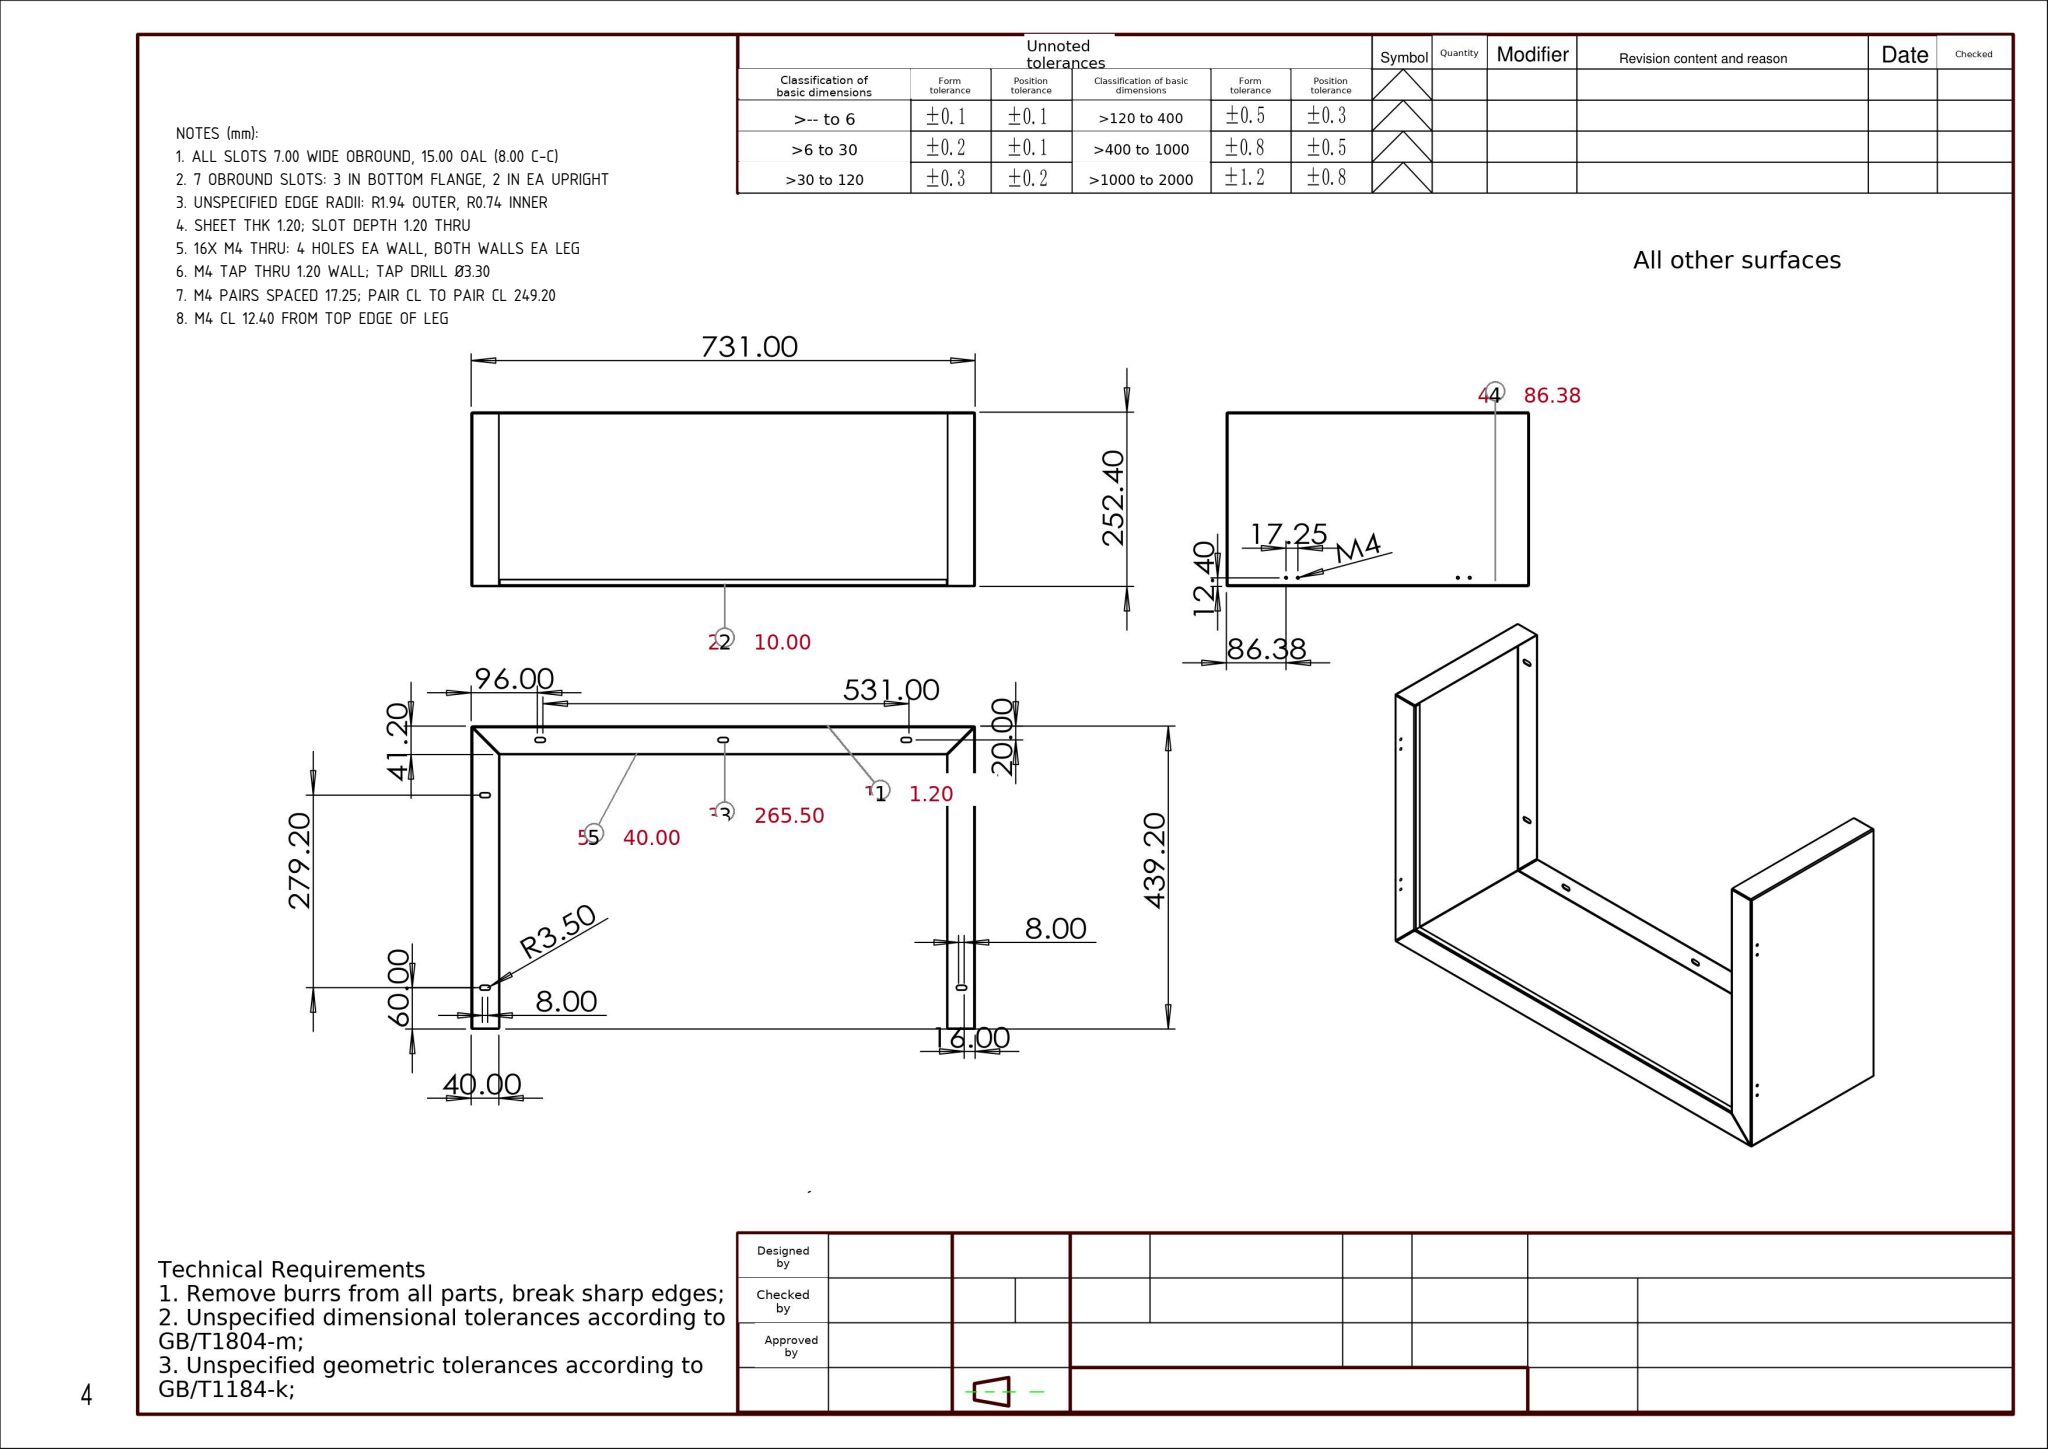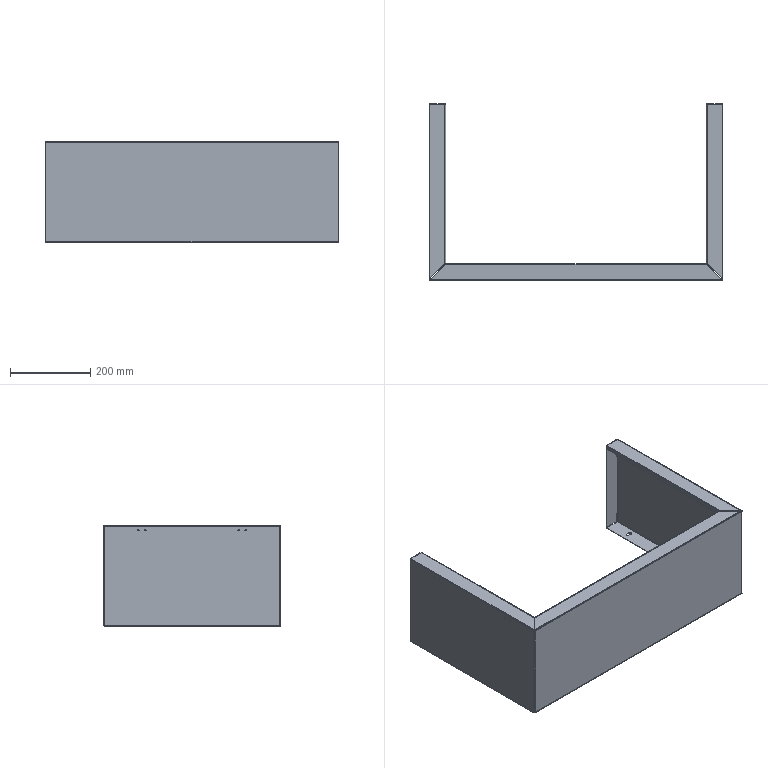Part | SolidWorks | mm | 1 solid | 185 faces | box 731 x 439.2 x 252.4 mm | volume 663802 mm3 | plane 114 | cylinder 63 | spline 8 | commonest cylinder face diameters 7 x21 3.3 x16 3.873 x13 1.473 x13
Drawing notes:
ALL SLOTS 7.00 WIDE OBROUND, 15.00 OAL (8.00 C-C) | from the solid: Ø7.00 z-axis cyl pairs 8.00 apart, e.g. x=96.01 & 104.01 at y=20.01; depth 1.2
7 OBROUND SLOTS: 3 IN BOTTOM FLANGE, 2 IN EA UPRIGHT | from the solid: Ø7.00 pairs: y=20.01 at x=96/104, 361.5/369.5, 627/635; x=16/24 and x=707/715 at y=100.01 & 379.21
UNSPECIFIED EDGE RADII: R1.94 OUTER, R0.74 INNER | from the solid: Edge cylinders Ø3.873 (R1.94) and Ø1.473 (R0.74) along all bbox edges
SHEET THK 1.20; SLOT DEPTH 1.20 THRU | from the solid: Planes x=0.01/1.21, z=0.01/1.21, z=251.21/252.41; Ø7.00 and Ø3.3 cyl length 1.2
16X M4 THRU: 4 HOLES EA WALL, BOTH WALLS EA LEG | from the solid: Ø3.3 x-axis holes len 1.2 at y=86.39,103.64,335.59,352.84 z=240.01, count 4 each = 16
M4 TAP THRU 1.20 WALL; TAP DRILL Ø3.30 | from the solid: Ø3.3 cylinders length 1.20 = wall thk (x planes 0.01-1.21, 40.01-41.21)
M4 PAIRS SPACED 17.25; PAIR CL TO PAIR CL 249.20 | from the solid: y=86.39 & 103.64, 335.59 & 352.84 (deltas 17.25; 335.59-86.39=249.20)
M4 CL 12.40 FROM TOP EDGE OF LEG | from the solid: hole z=240.01, part top z=252.41 -> 12.40